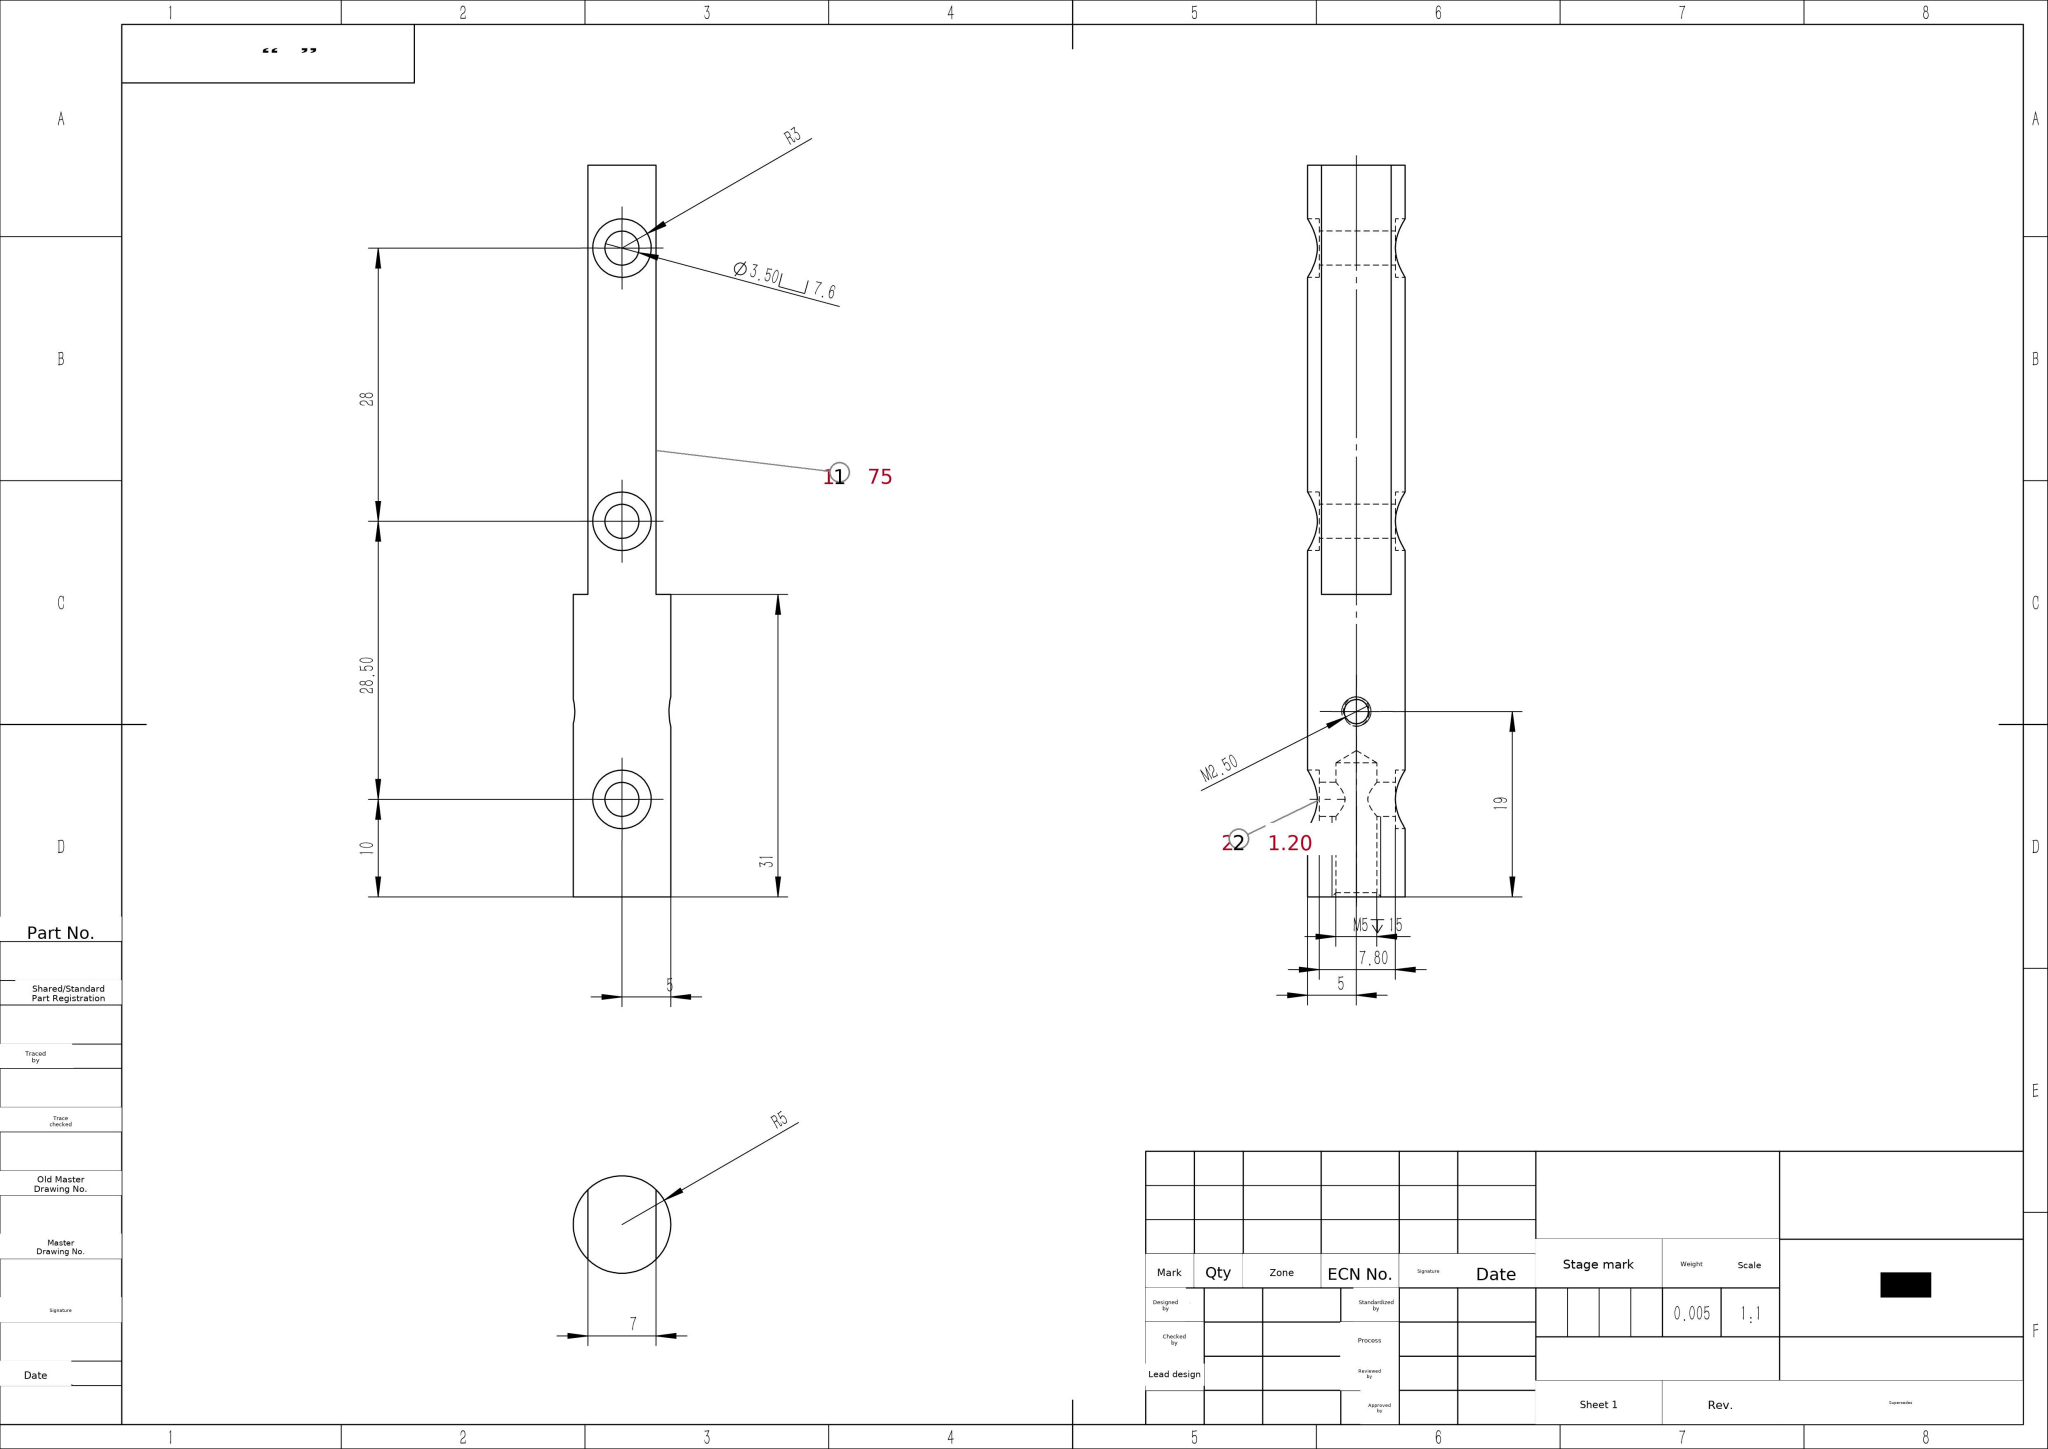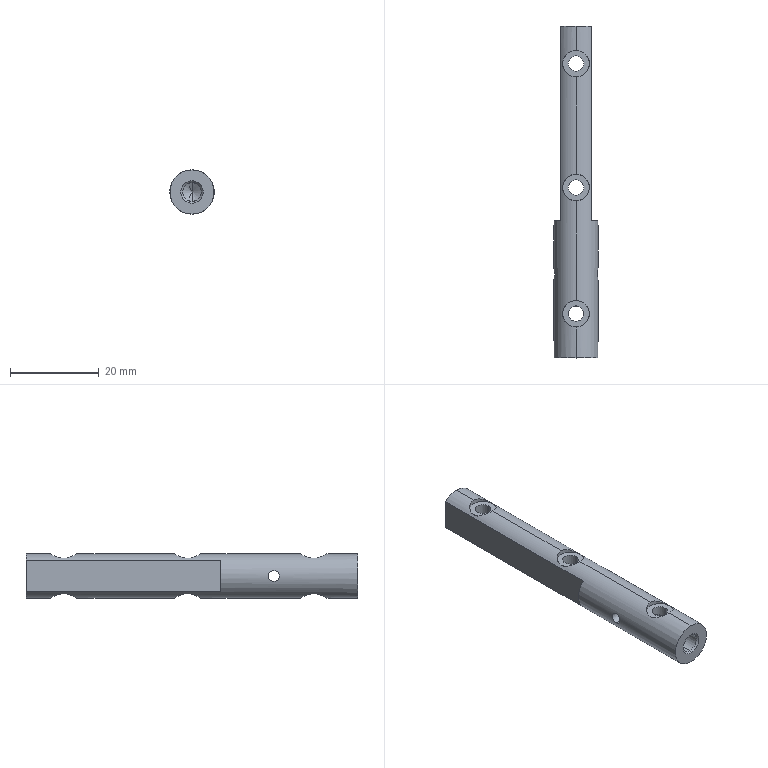Part | SolidWorks | mm | 1 solid | 44 faces | box 10 x 75 x 10 mm | volume 4659 mm3 | cylinder 26 | plane 12 | cone 6 | commonest cylinder face diameters 6 x12 3.5 x8 4.2 x2 2.5 x2 10 x2
build123d program:
from build123d import *

# Parameters (mm, degrees)
SKETCH1_R                   = 5
BOSS_EXTRUDE1_DEPTH         = 75
SKETCH2_W                   = 1.5
SKETCH2_H                   = 44
CUT_EXTRUDE1_DEPTH          = 37.5
SKETCH3_4_R                 = 1.75
CUT_EXTRUDE2_DEPTH          = 37.5
CUT_EXTRUDE3_START          = -3.8
SKETCH3_3_R                 = 3
SKETCH3_3_R_2               = 1.75
CUT_EXTRUDE3_DEPTH          = 75
CUT_EXTRUDE4_START          = 79
SKETCH3_4_2_R               = 3
SKETCH3_4_2_R_2             = 1.75
CUT_EXTRUDE4_DEPTH          = 75
M3_TAPPED_HOLE1_D           = 2.5
M3_TAPPED_HOLE1_CSINK_D     = 3.05
M3_TAPPED_HOLE1_CSINK_ANGLE = 90
M5_TAPPED_HOLE1_D           = 4.2
M5_TAPPED_HOLE1_DEPTH       = 13.738
M5_TAPPED_HOLE1_CSINK_D     = 5.05
M5_TAPPED_HOLE1_CSINK_ANGLE = 90
M5_TAPPED_HOLE1_TIP         = 1.262


with BuildPart() as part:
    # Sketch1 → Boss-Extrude1 (new body)
    with BuildSketch(Plane(origin=(0, 0, 0), x_dir=(1, 0, 0), z_dir=(0, 1, 0))):
        with Locations(Location((0, 0, 0), (0, 0, 270))):
            Circle(SKETCH1_R)
    extrude(amount=BOSS_EXTRUDE1_DEPTH)

    # Sketch2 → Cut-Extrude1 (cut, symmetric)
    with BuildSketch(Plane.XY):
        with Locations((-4.25, 53)):
            Rectangle(SKETCH2_W, SKETCH2_H)
        with Locations((4.25, 53)):
            Rectangle(SKETCH2_W, SKETCH2_H)
    extrude(amount=CUT_EXTRUDE1_DEPTH, both=True, mode=Mode.SUBTRACT)

    # Sketch3_4 → Cut-Extrude2 (cut, symmetric)
    with BuildSketch(Plane.XY):
        with Locations((0, 66.5)):
            Circle(SKETCH3_4_R)
        with Locations((0, 38.5)):
            Circle(SKETCH3_4_R)
        with Locations((0, 10)):
            Circle(SKETCH3_4_R)
    extrude(amount=CUT_EXTRUDE2_DEPTH, both=True, mode=Mode.SUBTRACT)

    # Sketch3_3 → Cut-Extrude3 (cut)
    # profile 1 of 3: a face of its own
    with BuildSketch(Plane.XY.offset(CUT_EXTRUDE3_START)):
        with Locations((0, 66.5)):
            Circle(SKETCH3_3_R)
        with Locations((0, 66.5)):
            Circle(SKETCH3_3_R_2, mode=Mode.SUBTRACT)
    # profile 2 of 3: a face of its own
    with BuildSketch(Plane.XY.offset(CUT_EXTRUDE3_START)):
        with Locations((0, 38.5)):
            Circle(SKETCH3_3_R)
        with Locations((0, 38.5)):
            Circle(SKETCH3_3_R_2, mode=Mode.SUBTRACT)
    # profile 3 of 3: a face of its own
    with BuildSketch(Plane.XY.offset(CUT_EXTRUDE3_START)):
        with Locations((0, 10)):
            Circle(SKETCH3_3_R)
        with Locations((0, 10)):
            Circle(SKETCH3_3_R_2, mode=Mode.SUBTRACT)
    extrude(amount=-CUT_EXTRUDE3_DEPTH, mode=Mode.SUBTRACT)

    # Sketch3_4 2 → Cut-Extrude4 (cut)
    # profile 1 of 3: a face of its own
    with BuildSketch(Plane.XY.offset(CUT_EXTRUDE4_START)):
        with Locations((0, 66.5)):
            Circle(SKETCH3_4_2_R)
        with Locations((0, 66.5)):
            Circle(SKETCH3_4_2_R_2, mode=Mode.SUBTRACT)
    # profile 2 of 3: a face of its own
    with BuildSketch(Plane.XY.offset(CUT_EXTRUDE4_START)):
        with Locations((0, 38.5)):
            Circle(SKETCH3_4_2_R)
        with Locations((0, 38.5)):
            Circle(SKETCH3_4_2_R_2, mode=Mode.SUBTRACT)
    # profile 3 of 3: a face of its own
    with BuildSketch(Plane.XY.offset(CUT_EXTRUDE4_START)):
        with Locations((0, 10)):
            Circle(SKETCH3_4_2_R)
        with Locations((0, 10)):
            Circle(SKETCH3_4_2_R_2, mode=Mode.SUBTRACT)
    extrude(amount=-CUT_EXTRUDE4_DEPTH, mode=Mode.SUBTRACT)

    # M3 Tapped Hole1 (through all)
    with Locations(Plane(origin=(5, 0, 0), x_dir=(0, 0, -1), z_dir=(1, 0, 0))):
        with Locations((0, 19)):
            CounterSinkHole(M3_TAPPED_HOLE1_D / 2, M3_TAPPED_HOLE1_CSINK_D / 2, counter_sink_angle=M3_TAPPED_HOLE1_CSINK_ANGLE)

    # M5 Tapped Hole1
    with Locations(Plane(origin=(0, 0, 0), x_dir=(-1, 0, 0), z_dir=(0, -1, 0))):
        with Locations((0, 0)):
            CounterSinkHole(M5_TAPPED_HOLE1_D / 2, M5_TAPPED_HOLE1_CSINK_D / 2, depth=M5_TAPPED_HOLE1_DEPTH, counter_sink_angle=M5_TAPPED_HOLE1_CSINK_ANGLE)
            with Locations((0, 0, -(M5_TAPPED_HOLE1_DEPTH + M5_TAPPED_HOLE1_TIP / 2))):  # 118° drill point
                Cone(0, M5_TAPPED_HOLE1_D / 2, M5_TAPPED_HOLE1_TIP, mode=Mode.SUBTRACT)


solid = part.part